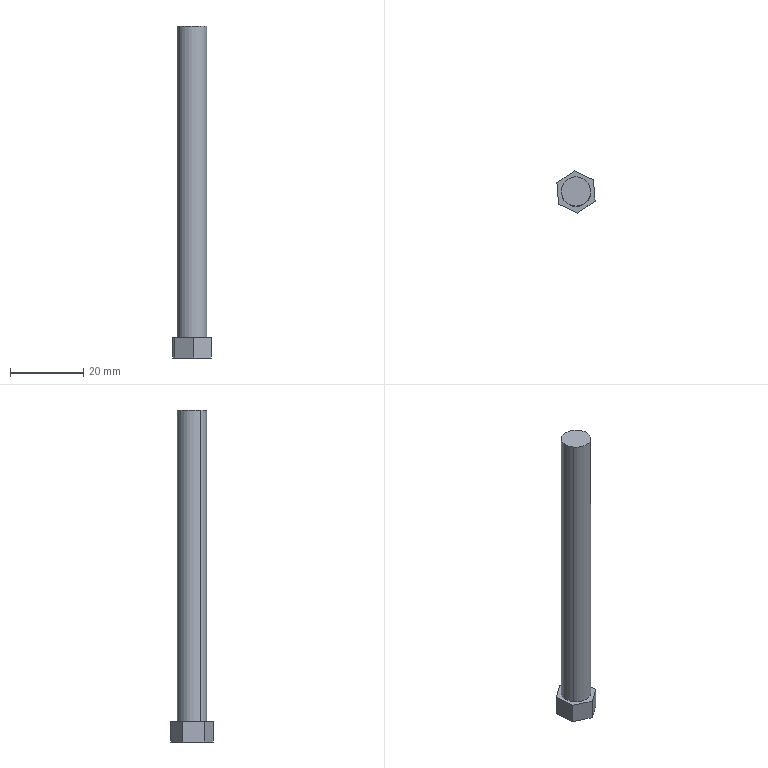Component | SolidWorks | 8Bolt85-1 | 1 solid | 11 faces | box 10.44 x 11.51 x 90.5 mm | volume 4749 mm3 | plane 9 | cylinder 2 | commonest cylinder face diameters 8 x2
STEP:
#1=CARTESIAN_POINT('',(3.855,4.242,4.48));
#2=VERTEX_POINT('',#1);
#3=CARTESIAN_POINT('',(3.596,4.063,4.48));
#4=VERTEX_POINT('',#3);
#5=CARTESIAN_POINT('',(3.725,4.152,4.48));
#6=DIRECTION('',(0.,0.,1.));
#7=DIRECTION('',(0.8216,0.5701,0.));
#8=AXIS2_PLACEMENT_3D('',#5,#6,#7);
#9=CIRCLE('',#8,0.1575);
#10=EDGE_CURVE('',#2,#4,#9,.T.);
#11=ORIENTED_EDGE('',*,*,#10,.F.);
#12=CARTESIAN_POINT('',(3.855,4.242,1.133));
#13=VERTEX_POINT('',#12);
#14=CARTESIAN_POINT('',(3.855,4.242,4.48));
#15=DIRECTION('',(0.,0.,-1.));
#16=VECTOR('',#15,39.37);
#17=LINE('',#14,#16);
#18=EDGE_CURVE('',#2,#13,#17,.T.);
#19=ORIENTED_EDGE('',*,*,#18,.T.);
#20=CARTESIAN_POINT('',(3.596,4.063,1.133));
#21=VERTEX_POINT('',#20);
#22=CARTESIAN_POINT('',(3.725,4.152,1.133));
#23=DIRECTION('',(0.,0.,1.));
#24=DIRECTION('',(0.8216,0.5701,0.));
#25=AXIS2_PLACEMENT_3D('',#22,#23,#24);
#26=CIRCLE('',#25,0.1575);
#27=EDGE_CURVE('',#13,#21,#26,.T.);
#28=ORIENTED_EDGE('',*,*,#27,.T.);
#29=CARTESIAN_POINT('',(3.596,4.063,4.48));
#30=DIRECTION('',(0.,0.,-1.));
#31=VECTOR('',#30,39.37);
#32=LINE('',#29,#31);
#33=EDGE_CURVE('',#4,#21,#32,.T.);
#34=ORIENTED_EDGE('',*,*,#33,.F.);
#35=EDGE_LOOP('',(#11,#19,#28,#34));
#36=FACE_OUTER_BOUND('',#35,.T.);
#37=CARTESIAN_POINT('',(3.725,4.152,4.48));
#38=DIRECTION('',(0.,0.,-1.));
#39=DIRECTION('',(-0.8216,-0.5701,0.));
#40=AXIS2_PLACEMENT_3D('',#37,#38,#39);
#41=CYLINDRICAL_SURFACE('',#40,0.1575);
#42=ADVANCED_FACE('',(#36),#41,.T.);
#43=CARTESIAN_POINT('',(3.931,4.055,0.9168));
#44=VERTEX_POINT('',#43);
#45=CARTESIAN_POINT('',(3.912,4.282,0.9168));
#46=VERTEX_POINT('',#45);
#47=CARTESIAN_POINT('',(3.931,4.055,0.9168));
#48=DIRECTION('',(-0.08293,0.9966,0.));
#49=VECTOR('',#48,39.37);
#50=LINE('',#47,#49);
#51=EDGE_CURVE('',#44,#46,#50,.T.);
#52=ORIENTED_EDGE('',*,*,#51,.T.);
#53=CARTESIAN_POINT('',(3.912,4.282,1.133));
#54=VERTEX_POINT('',#53);
#55=CARTESIAN_POINT('',(3.912,4.282,1.133));
#56=DIRECTION('',(0.,0.,-1.));
#57=VECTOR('',#56,39.37);
#58=LINE('',#55,#57);
#59=EDGE_CURVE('',#54,#46,#58,.T.);
#60=ORIENTED_EDGE('',*,*,#59,.F.);
#61=CARTESIAN_POINT('',(3.931,4.055,1.133));
#62=VERTEX_POINT('',#61);
#63=CARTESIAN_POINT('',(3.931,4.055,1.133));
#64=DIRECTION('',(-0.08293,0.9966,0.));
#65=VECTOR('',#64,39.37);
#66=LINE('',#63,#65);
#67=EDGE_CURVE('',#62,#54,#66,.T.);
#68=ORIENTED_EDGE('',*,*,#67,.F.);
#69=CARTESIAN_POINT('',(3.931,4.055,1.133));
#70=DIRECTION('',(0.,0.,-1.));
#71=VECTOR('',#70,39.37);
#72=LINE('',#69,#71);
#73=EDGE_CURVE('',#62,#44,#72,.T.);
#74=ORIENTED_EDGE('',*,*,#73,.T.);
#75=EDGE_LOOP('',(#52,#60,#68,#74));
#76=FACE_OUTER_BOUND('',#75,.T.);
#77=CARTESIAN_POINT('',(3.931,4.055,1.133));
#78=DIRECTION('',(-0.9966,-0.08293,0.));
#79=DIRECTION('',(0.08293,-0.9966,0.));
#80=AXIS2_PLACEMENT_3D('',#77,#78,#79);
#81=PLANE('',#80);
#82=ADVANCED_FACE('',(#76),#81,.F.);
#83=CARTESIAN_POINT('',(3.706,4.379,0.9168));
#84=VERTEX_POINT('',#83);
#85=CARTESIAN_POINT('',(3.912,4.282,0.9168));
#86=DIRECTION('',(-0.9045,0.4265,0.));
#87=VECTOR('',#86,39.37);
#88=LINE('',#85,#87);
#89=EDGE_CURVE('',#46,#84,#88,.T.);
#90=ORIENTED_EDGE('',*,*,#89,.T.);
#91=CARTESIAN_POINT('',(3.706,4.379,1.133));
#92=VERTEX_POINT('',#91);
#93=CARTESIAN_POINT('',(3.706,4.379,1.133));
#94=DIRECTION('',(0.,0.,-1.));
#95=VECTOR('',#94,39.37);
#96=LINE('',#93,#95);
#97=EDGE_CURVE('',#92,#84,#96,.T.);
#98=ORIENTED_EDGE('',*,*,#97,.F.);
#99=CARTESIAN_POINT('',(3.912,4.282,1.133));
#100=DIRECTION('',(-0.9045,0.4265,0.));
#101=VECTOR('',#100,39.37);
#102=LINE('',#99,#101);
#103=EDGE_CURVE('',#54,#92,#102,.T.);
#104=ORIENTED_EDGE('',*,*,#103,.F.);
#105=ORIENTED_EDGE('',*,*,#59,.T.);
#106=EDGE_LOOP('',(#90,#98,#104,#105));
#107=FACE_OUTER_BOUND('',#106,.T.);
#108=CARTESIAN_POINT('',(3.912,4.282,1.133));
#109=DIRECTION('',(-0.4265,-0.9045,0.));
#110=DIRECTION('',(0.9045,-0.4265,0.));
#111=AXIS2_PLACEMENT_3D('',#108,#109,#110);
#112=PLANE('',#111);
#113=ADVANCED_FACE('',(#107),#112,.F.);
#114=CARTESIAN_POINT('',(3.52,4.249,0.9168));
#115=VERTEX_POINT('',#114);
#116=CARTESIAN_POINT('',(3.706,4.379,0.9168));
#117=DIRECTION('',(-0.8216,-0.5701,0.));
#118=VECTOR('',#117,39.37);
#119=LINE('',#116,#118);
#120=EDGE_CURVE('',#84,#115,#119,.T.);
#121=ORIENTED_EDGE('',*,*,#120,.T.);
#122=CARTESIAN_POINT('',(3.52,4.249,1.133));
#123=VERTEX_POINT('',#122);
#124=CARTESIAN_POINT('',(3.52,4.249,1.133));
#125=DIRECTION('',(0.,0.,-1.));
#126=VECTOR('',#125,39.37);
#127=LINE('',#124,#126);
#128=EDGE_CURVE('',#123,#115,#127,.T.);
#129=ORIENTED_EDGE('',*,*,#128,.F.);
#130=CARTESIAN_POINT('',(3.706,4.379,1.133));
#131=DIRECTION('',(-0.8216,-0.5701,0.));
#132=VECTOR('',#131,39.37);
#133=LINE('',#130,#132);
#134=EDGE_CURVE('',#92,#123,#133,.T.);
#135=ORIENTED_EDGE('',*,*,#134,.F.);
#136=ORIENTED_EDGE('',*,*,#97,.T.);
#137=EDGE_LOOP('',(#121,#129,#135,#136));
#138=FACE_OUTER_BOUND('',#137,.T.);
#139=CARTESIAN_POINT('',(3.706,4.379,1.133));
#140=DIRECTION('',(0.5701,-0.8216,0.));
#141=DIRECTION('',(0.,0.,-1.));
#142=AXIS2_PLACEMENT_3D('',#139,#140,#141);
#143=PLANE('',#142);
#144=ADVANCED_FACE('',(#138),#143,.F.);
#145=CARTESIAN_POINT('',(3.538,4.023,0.9168));
#146=VERTEX_POINT('',#145);
#147=CARTESIAN_POINT('',(3.52,4.249,0.9168));
#148=DIRECTION('',(0.08293,-0.9966,0.));
#149=VECTOR('',#148,39.37);
#150=LINE('',#147,#149);
#151=EDGE_CURVE('',#115,#146,#150,.T.);
#152=ORIENTED_EDGE('',*,*,#151,.T.);
#153=CARTESIAN_POINT('',(3.538,4.023,1.133));
#154=VERTEX_POINT('',#153);
#155=CARTESIAN_POINT('',(3.538,4.023,1.133));
#156=DIRECTION('',(0.,0.,-1.));
#157=VECTOR('',#156,39.37);
#158=LINE('',#155,#157);
#159=EDGE_CURVE('',#154,#146,#158,.T.);
#160=ORIENTED_EDGE('',*,*,#159,.F.);
#161=CARTESIAN_POINT('',(3.52,4.249,1.133));
#162=DIRECTION('',(0.08293,-0.9966,0.));
#163=VECTOR('',#162,39.37);
#164=LINE('',#161,#163);
#165=EDGE_CURVE('',#123,#154,#164,.T.);
#166=ORIENTED_EDGE('',*,*,#165,.F.);
#167=ORIENTED_EDGE('',*,*,#128,.T.);
#168=EDGE_LOOP('',(#152,#160,#166,#167));
#169=FACE_OUTER_BOUND('',#168,.T.);
#170=CARTESIAN_POINT('',(3.52,4.249,1.133));
#171=DIRECTION('',(0.9966,0.08293,0.));
#172=DIRECTION('',(-0.08293,0.9966,0.));
#173=AXIS2_PLACEMENT_3D('',#170,#171,#172);
#174=PLANE('',#173);
#175=ADVANCED_FACE('',(#169),#174,.F.);
#176=CARTESIAN_POINT('',(3.744,3.926,0.9168));
#177=VERTEX_POINT('',#176);
#178=CARTESIAN_POINT('',(3.538,4.023,0.9168));
#179=DIRECTION('',(0.9045,-0.4265,0.));
#180=VECTOR('',#179,39.37);
#181=LINE('',#178,#180);
#182=EDGE_CURVE('',#146,#177,#181,.T.);
#183=ORIENTED_EDGE('',*,*,#182,.T.);
#184=CARTESIAN_POINT('',(3.744,3.926,1.133));
#185=VERTEX_POINT('',#184);
#186=CARTESIAN_POINT('',(3.744,3.926,1.133));
#187=DIRECTION('',(0.,0.,-1.));
#188=VECTOR('',#187,39.37);
#189=LINE('',#186,#188);
#190=EDGE_CURVE('',#185,#177,#189,.T.);
#191=ORIENTED_EDGE('',*,*,#190,.F.);
#192=CARTESIAN_POINT('',(3.538,4.023,1.133));
#193=DIRECTION('',(0.9045,-0.4265,0.));
#194=VECTOR('',#193,39.37);
#195=LINE('',#192,#194);
#196=EDGE_CURVE('',#154,#185,#195,.T.);
#197=ORIENTED_EDGE('',*,*,#196,.F.);
#198=ORIENTED_EDGE('',*,*,#159,.T.);
#199=EDGE_LOOP('',(#183,#191,#197,#198));
#200=FACE_OUTER_BOUND('',#199,.T.);
#201=CARTESIAN_POINT('',(3.538,4.023,1.133));
#202=DIRECTION('',(0.4265,0.9045,0.));
#203=DIRECTION('',(-0.9045,0.4265,0.));
#204=AXIS2_PLACEMENT_3D('',#201,#202,#203);
#205=PLANE('',#204);
#206=ADVANCED_FACE('',(#200),#205,.F.);
#207=CARTESIAN_POINT('',(3.744,3.926,0.9168));
#208=DIRECTION('',(0.8216,0.5701,0.));
#209=VECTOR('',#208,39.37);
#210=LINE('',#207,#209);
#211=EDGE_CURVE('',#177,#44,#210,.T.);
#212=ORIENTED_EDGE('',*,*,#211,.T.);
#213=ORIENTED_EDGE('',*,*,#73,.F.);
#214=CARTESIAN_POINT('',(3.744,3.926,1.133));
#215=DIRECTION('',(0.8216,0.5701,0.));
#216=VECTOR('',#215,39.37);
#217=LINE('',#214,#216);
#218=EDGE_CURVE('',#185,#62,#217,.T.);
#219=ORIENTED_EDGE('',*,*,#218,.F.);
#220=ORIENTED_EDGE('',*,*,#190,.T.);
#221=EDGE_LOOP('',(#212,#213,#219,#220));
#222=FACE_OUTER_BOUND('',#221,.T.);
#223=CARTESIAN_POINT('',(3.744,3.926,1.133));
#224=DIRECTION('',(-0.5701,0.8216,0.));
#225=DIRECTION('',(-0.8216,-0.5701,0.));
#226=AXIS2_PLACEMENT_3D('',#223,#224,#225);
#227=PLANE('',#226);
#228=ADVANCED_FACE('',(#222),#227,.F.);
#229=CARTESIAN_POINT('',(3.725,4.152,1.133));
#230=DIRECTION('',(0.,0.,1.));
#231=DIRECTION('',(0.8216,0.5701,0.));
#232=AXIS2_PLACEMENT_3D('',#229,#230,#231);
#233=CIRCLE('',#232,0.1575);
#234=EDGE_CURVE('',#21,#13,#233,.T.);
#235=ORIENTED_EDGE('',*,*,#234,.F.);
#236=ORIENTED_EDGE('',*,*,#27,.F.);
#237=EDGE_LOOP('',(#235,#236));
#238=FACE_BOUND('',#237,.T.);
#239=ORIENTED_EDGE('',*,*,#67,.T.);
#240=ORIENTED_EDGE('',*,*,#103,.T.);
#241=ORIENTED_EDGE('',*,*,#134,.T.);
#242=ORIENTED_EDGE('',*,*,#165,.T.);
#243=ORIENTED_EDGE('',*,*,#196,.T.);
#244=ORIENTED_EDGE('',*,*,#218,.T.);
#245=EDGE_LOOP('',(#239,#240,#241,#242,#243,#244));
#246=FACE_OUTER_BOUND('',#245,.T.);
#247=CARTESIAN_POINT('',(3.725,4.152,1.133));
#248=DIRECTION('',(0.,0.,1.));
#249=DIRECTION('',(0.8216,0.5701,0.));
#250=AXIS2_PLACEMENT_3D('',#247,#248,#249);
#251=PLANE('',#250);
#252=ADVANCED_FACE('',(#238,#246),#251,.T.);
#253=ORIENTED_EDGE('',*,*,#51,.F.);
#254=ORIENTED_EDGE('',*,*,#211,.F.);
#255=ORIENTED_EDGE('',*,*,#182,.F.);
#256=ORIENTED_EDGE('',*,*,#151,.F.);
#257=ORIENTED_EDGE('',*,*,#120,.F.);
#258=ORIENTED_EDGE('',*,*,#89,.F.);
#259=EDGE_LOOP('',(#253,#254,#255,#256,#257,#258));
#260=FACE_OUTER_BOUND('',#259,.T.);
#261=CARTESIAN_POINT('',(3.725,4.152,0.9168));
#262=DIRECTION('',(0.,0.,1.));
#263=DIRECTION('',(0.8216,0.5701,0.));
#264=AXIS2_PLACEMENT_3D('',#261,#262,#263);
#265=PLANE('',#264);
#266=ADVANCED_FACE('',(#260),#265,.F.);
#267=ORIENTED_EDGE('',*,*,#18,.F.);
#268=CARTESIAN_POINT('',(3.725,4.152,4.48));
#269=DIRECTION('',(0.,0.,1.));
#270=DIRECTION('',(0.8216,0.5701,0.));
#271=AXIS2_PLACEMENT_3D('',#268,#269,#270);
#272=CIRCLE('',#271,0.1575);
#273=EDGE_CURVE('',#4,#2,#272,.T.);
#274=ORIENTED_EDGE('',*,*,#273,.F.);
#275=ORIENTED_EDGE('',*,*,#33,.T.);
#276=ORIENTED_EDGE('',*,*,#234,.T.);
#277=EDGE_LOOP('',(#267,#274,#275,#276));
#278=FACE_OUTER_BOUND('',#277,.T.);
#279=CARTESIAN_POINT('',(3.725,4.152,4.48));
#280=DIRECTION('',(0.,0.,-1.));
#281=DIRECTION('',(-0.8216,-0.5701,0.));
#282=AXIS2_PLACEMENT_3D('',#279,#280,#281);
#283=CYLINDRICAL_SURFACE('',#282,0.1575);
#284=ADVANCED_FACE('',(#278),#283,.T.);
#285=ORIENTED_EDGE('',*,*,#273,.T.);
#286=ORIENTED_EDGE('',*,*,#10,.T.);
#287=EDGE_LOOP('',(#285,#286));
#288=FACE_OUTER_BOUND('',#287,.T.);
#289=CARTESIAN_POINT('',(3.725,4.152,4.48));
#290=DIRECTION('',(0.,0.,1.));
#291=DIRECTION('',(0.8216,0.5701,0.));
#292=AXIS2_PLACEMENT_3D('',#289,#290,#291);
#293=PLANE('',#292);
#294=ADVANCED_FACE('',(#288),#293,.T.);
#295=CLOSED_SHELL('',(#42,#82,#113,#144,#175,#206,#228,#252,#266,#284,#294));
#296=MANIFOLD_SOLID_BREP('',#295);
#297=CARTESIAN_POINT('',(0.,0.,0.));
#298=DIRECTION('',(0.,0.,1.));
#299=DIRECTION('',(1.,0.,0.));
#300=AXIS2_PLACEMENT_3D('',#297,#298,#299);
#301=(LENGTH_UNIT()NAMED_UNIT(*)SI_UNIT($,.METRE.));
#302=LENGTH_MEASURE_WITH_UNIT(LENGTH_MEASURE(0.0254),#301);
#303=DIMENSIONAL_EXPONENTS(1.,0.,0.,0.,0.,0.,0.);
#304=(CONVERSION_BASED_UNIT('',#302)LENGTH_UNIT()NAMED_UNIT(#303));
#305=UNCERTAINTY_MEASURE_WITH_UNIT(LENGTH_MEASURE(0.00001),#304,'','');
#306=(NAMED_UNIT(*)PLANE_ANGLE_UNIT()SI_UNIT($,.RADIAN.));
#307=(NAMED_UNIT(*)SI_UNIT($,.STERADIAN.)SOLID_ANGLE_UNIT());
#308=(GEOMETRIC_REPRESENTATION_CONTEXT(3)GLOBAL_UNCERTAINTY_ASSIGNED_CONTEXT((#305))GLOBAL_UNIT_ASSIGNED_CONTEXT((#304,#306,#307))REPRESENTATION_CONTEXT('',''));
#309=ADVANCED_BREP_SHAPE_REPRESENTATION('',(#296,#300),#308);
#310=COLOUR_RGB('',0.7922,0.8196,0.9333);
#311=FILL_AREA_STYLE_COLOUR('',#310);
#312=FILL_AREA_STYLE('',(#311));
#313=SURFACE_STYLE_FILL_AREA(#312);
#314=SURFACE_SIDE_STYLE('',(#313));
#315=SURFACE_STYLE_USAGE(.BOTH.,#314);
#316=PRESENTATION_STYLE_ASSIGNMENT((#315));
#317=STYLED_ITEM('',(#316),#296);
#318=PRESENTATION_LAYER_ASSIGNMENT('','',(#317));
#319=(LENGTH_UNIT()NAMED_UNIT(*)SI_UNIT($,.METRE.));
#320=LENGTH_MEASURE_WITH_UNIT(LENGTH_MEASURE(0.0254),#319);
#321=DIMENSIONAL_EXPONENTS(1.,0.,0.,0.,0.,0.,0.);
#322=(CONVERSION_BASED_UNIT('',#320)LENGTH_UNIT()NAMED_UNIT(#321));
#323=UNCERTAINTY_MEASURE_WITH_UNIT(LENGTH_MEASURE(0.00001),#322,'','');
#324=(NAMED_UNIT(*)PLANE_ANGLE_UNIT()SI_UNIT($,.RADIAN.));
#325=(NAMED_UNIT(*)SI_UNIT($,.STERADIAN.)SOLID_ANGLE_UNIT());
#326=(GEOMETRIC_REPRESENTATION_CONTEXT(3)GLOBAL_UNCERTAINTY_ASSIGNED_CONTEXT((#323))GLOBAL_UNIT_ASSIGNED_CONTEXT((#322,#324,#325))REPRESENTATION_CONTEXT('',''));
#327=MECHANICAL_DESIGN_GEOMETRIC_PRESENTATION_REPRESENTATION('',(#317),#326);